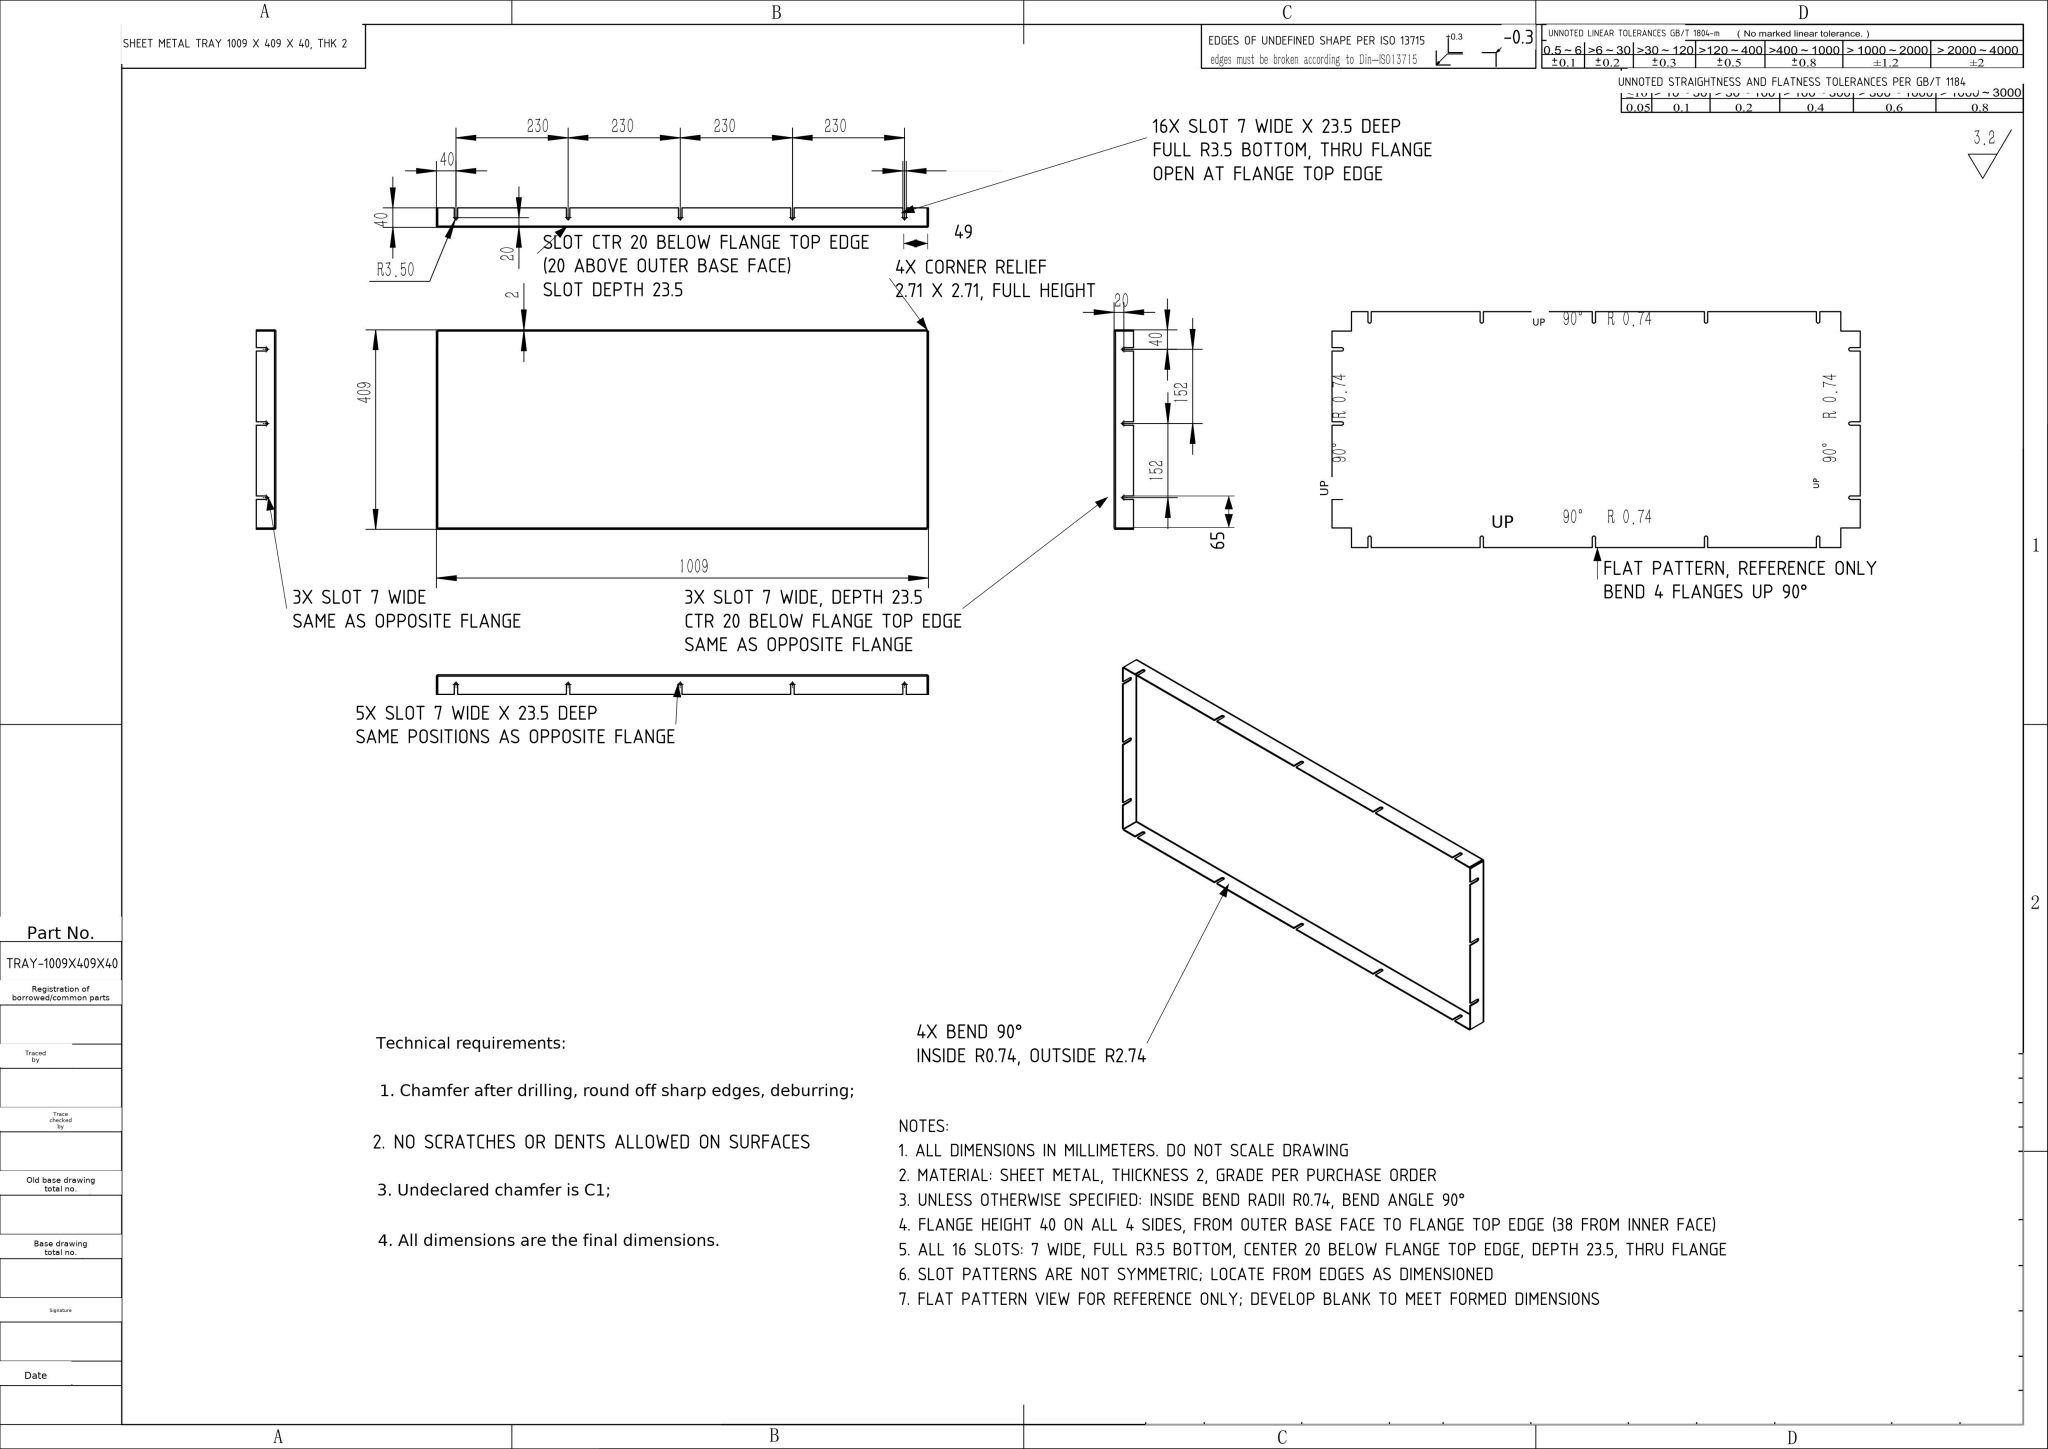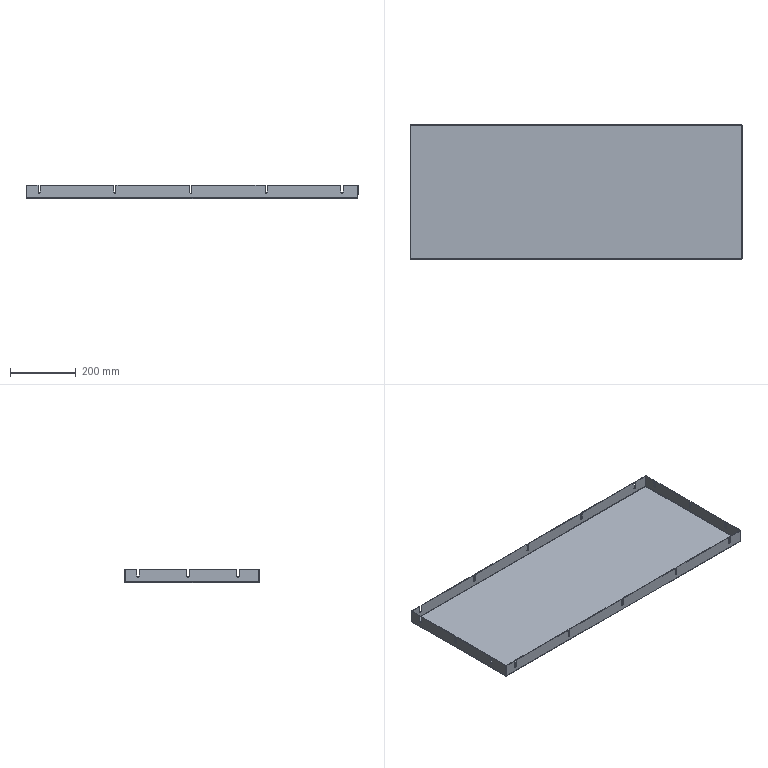Part | NX | mm | 1 solid | 112 faces | box 1009 x 409 x 40 mm | volume 1029902 mm3 | plane 70 | cylinder 34 | spline 8 | commonest cylinder face diameters 7 x26 5.473 x4 1.473 x4